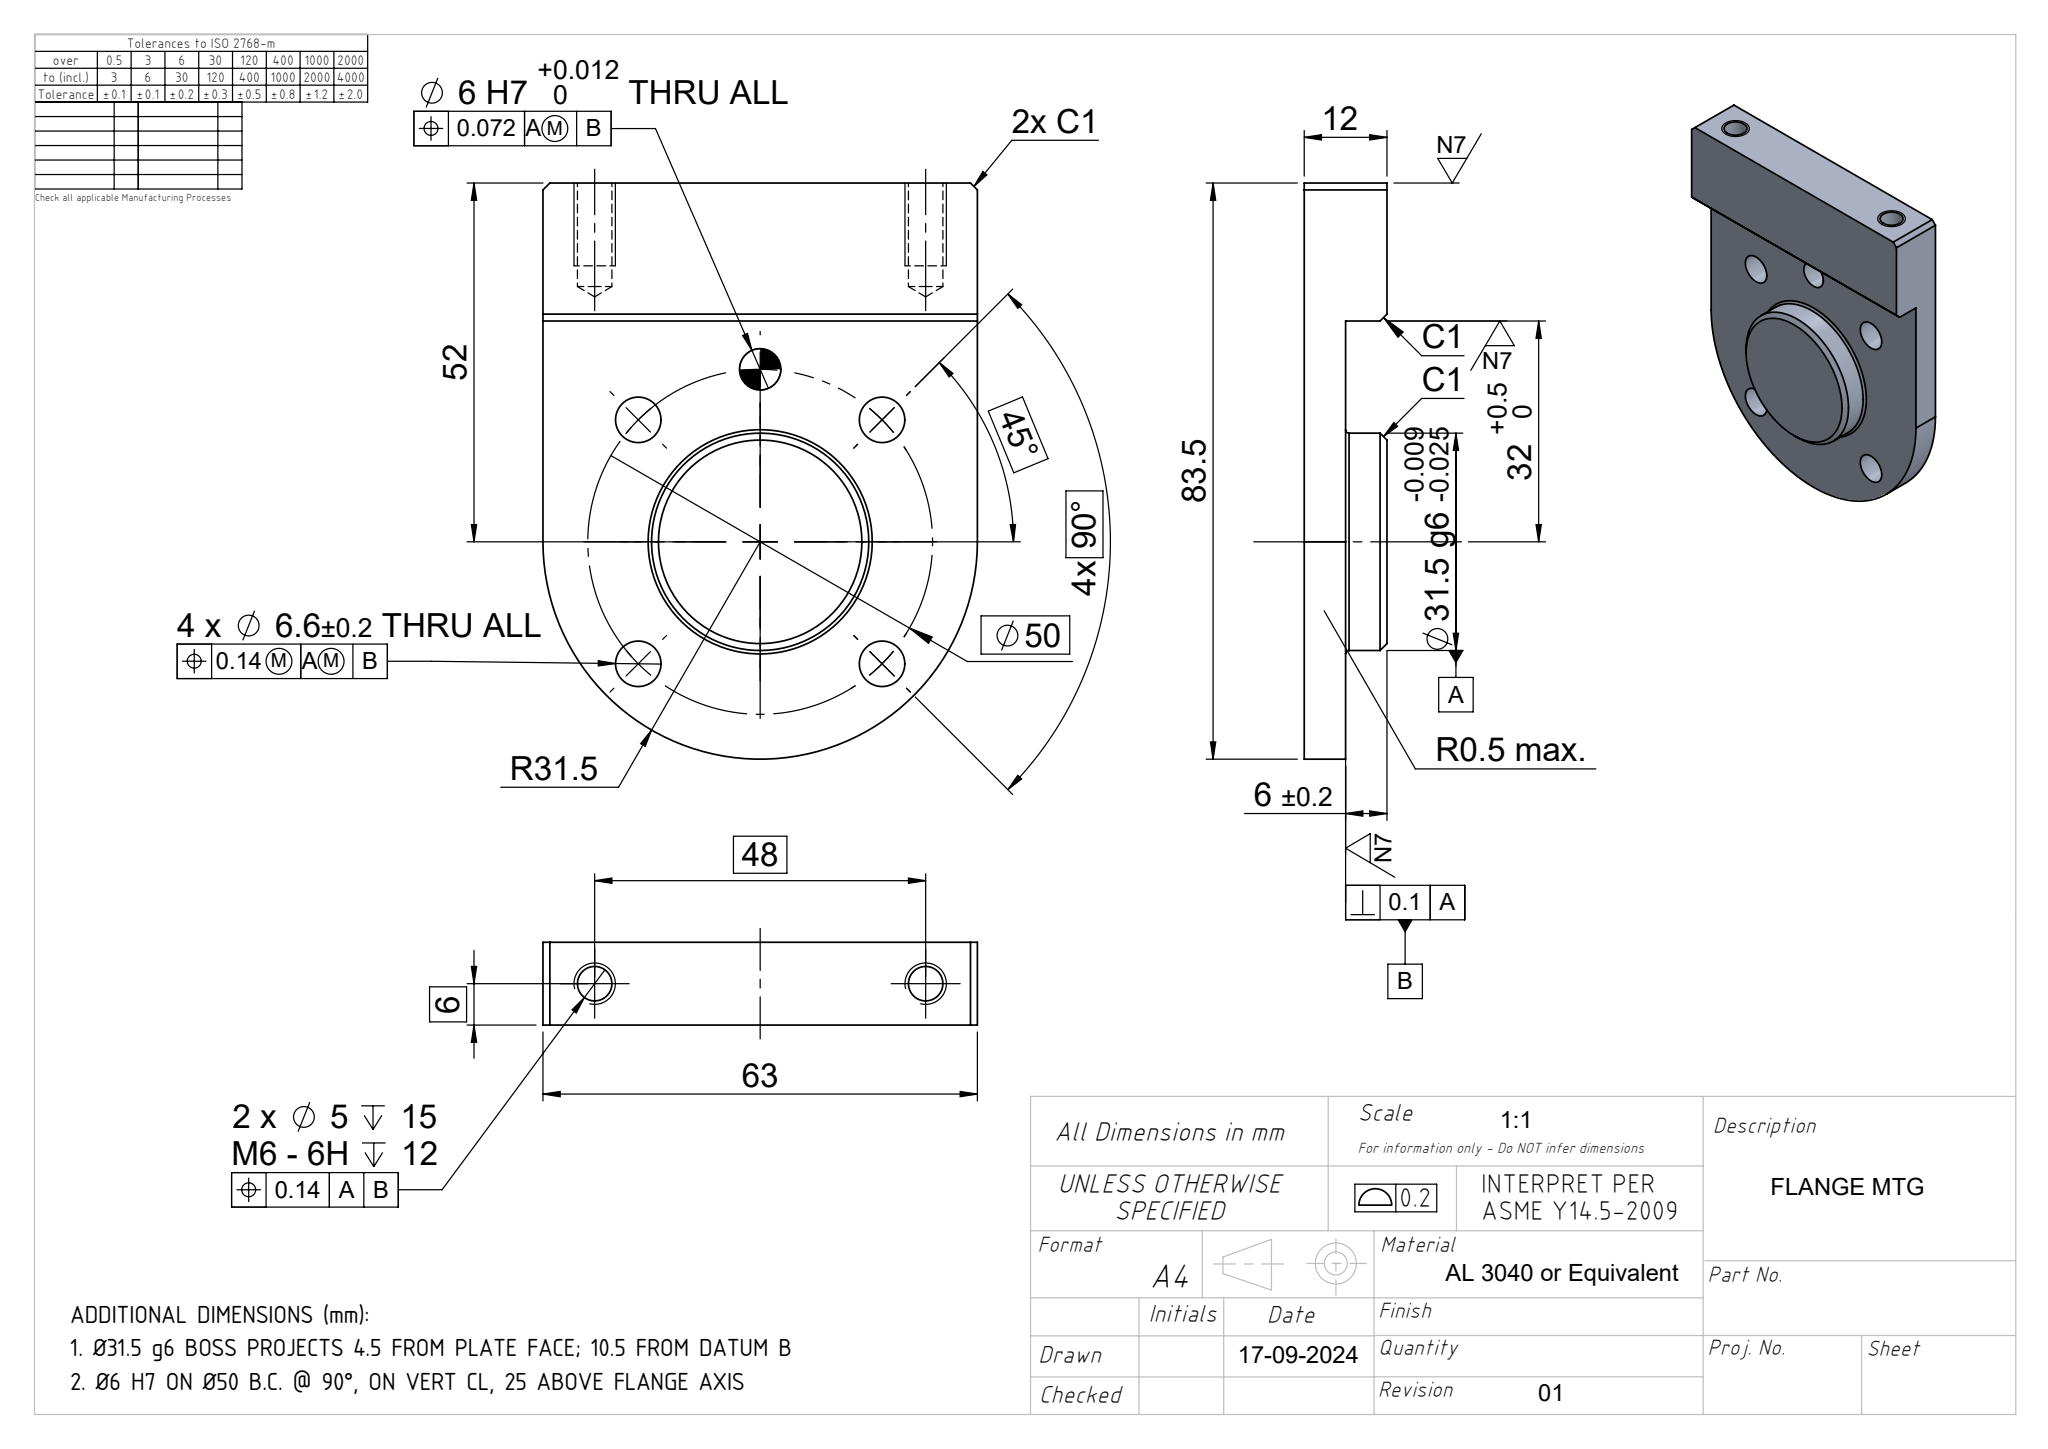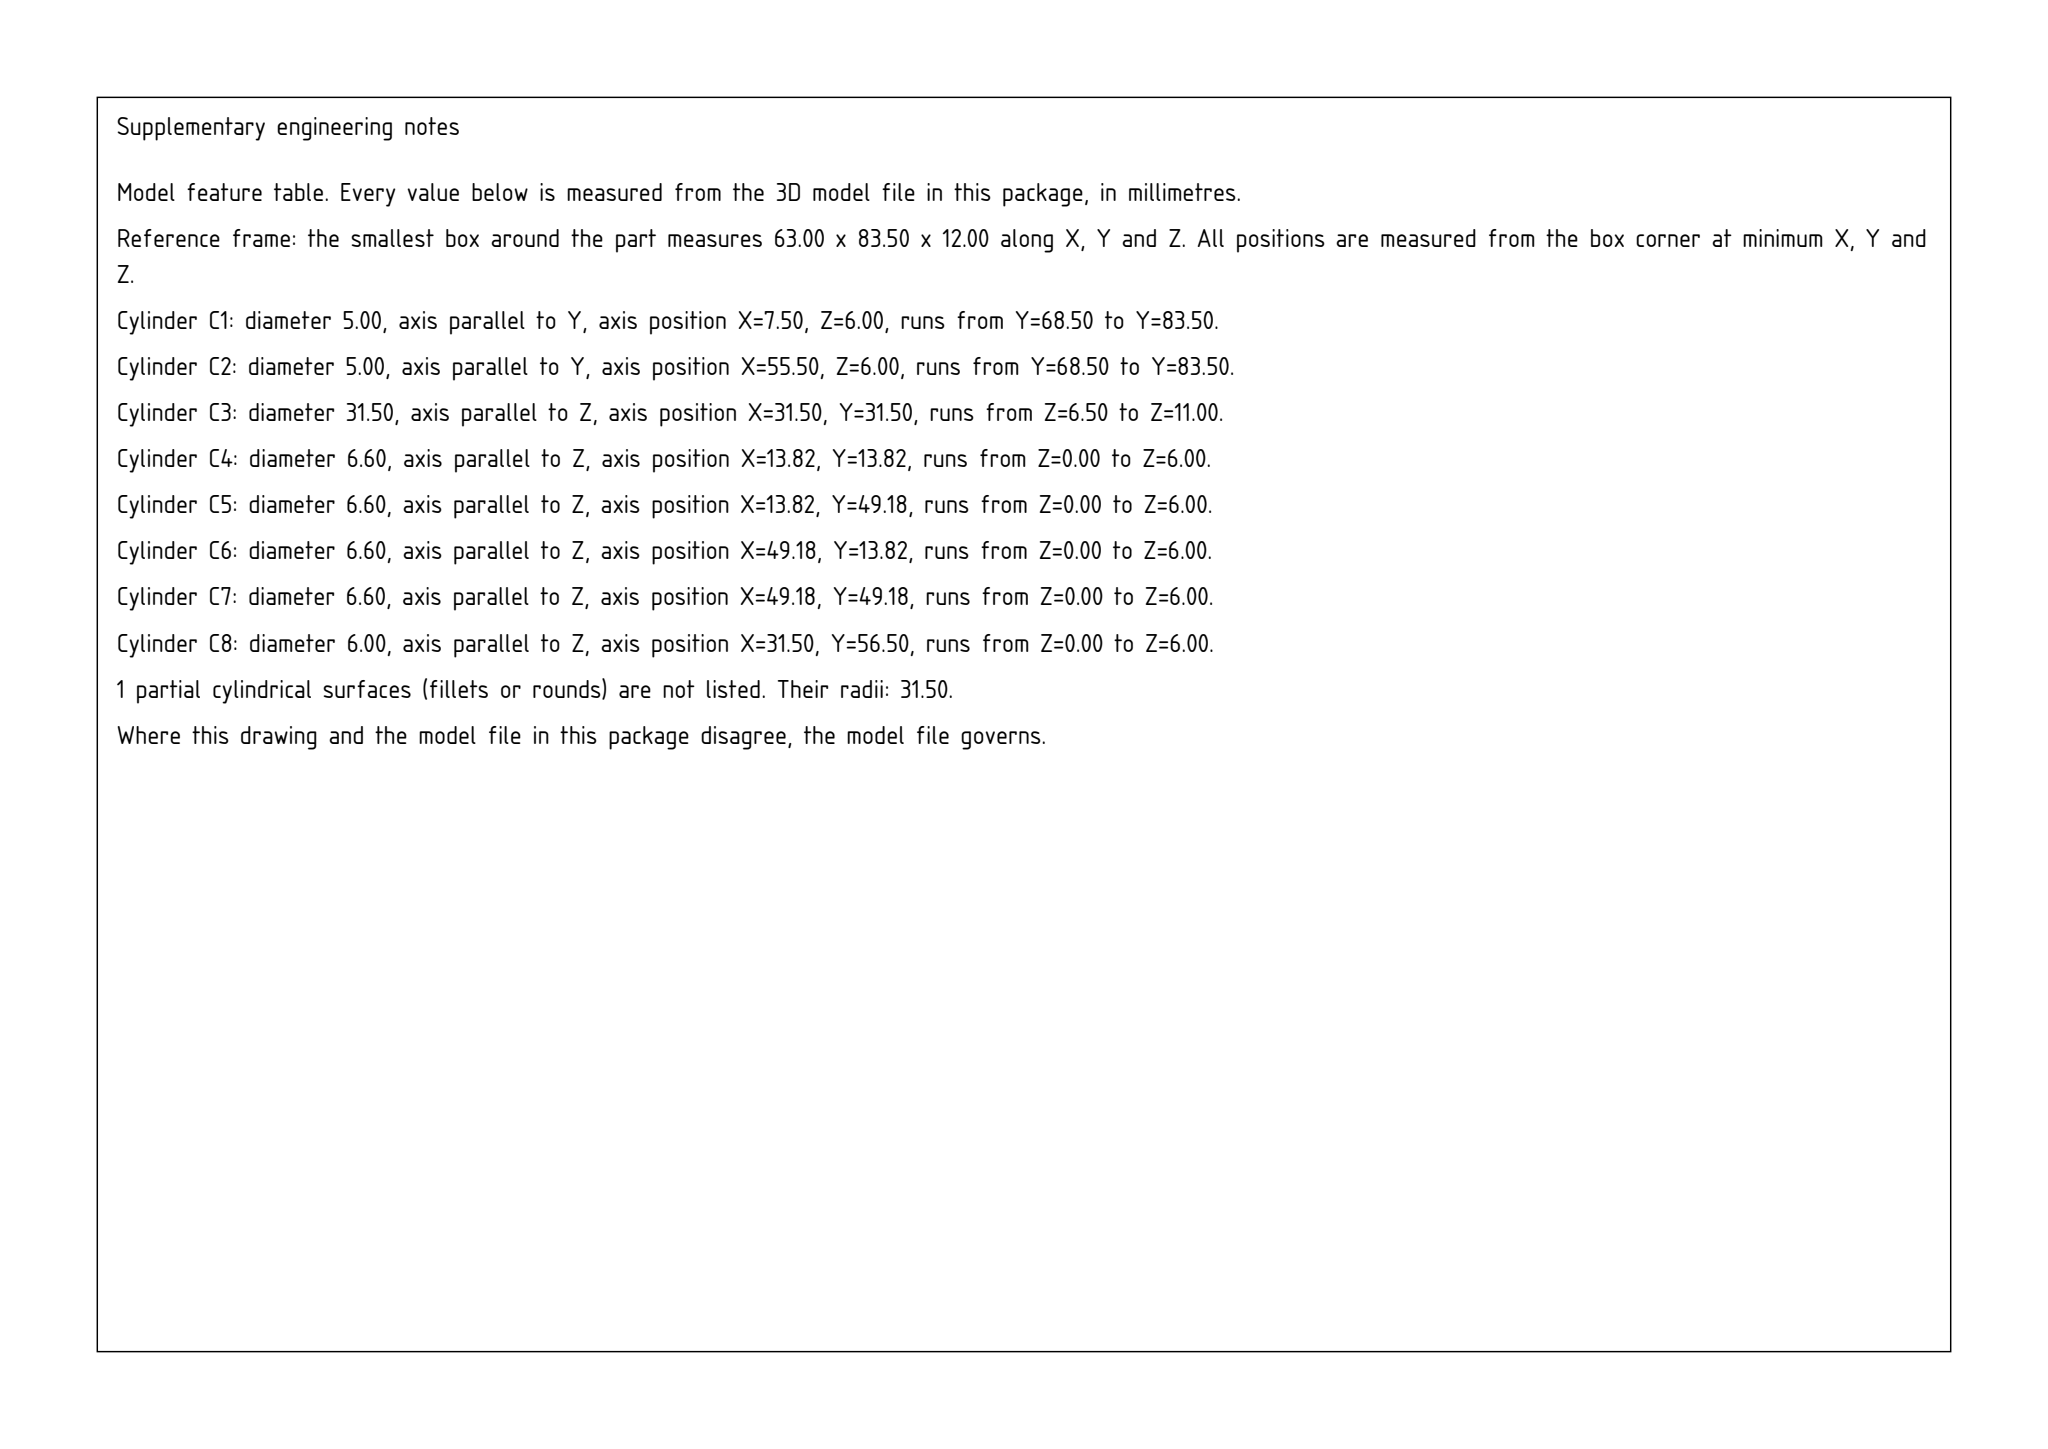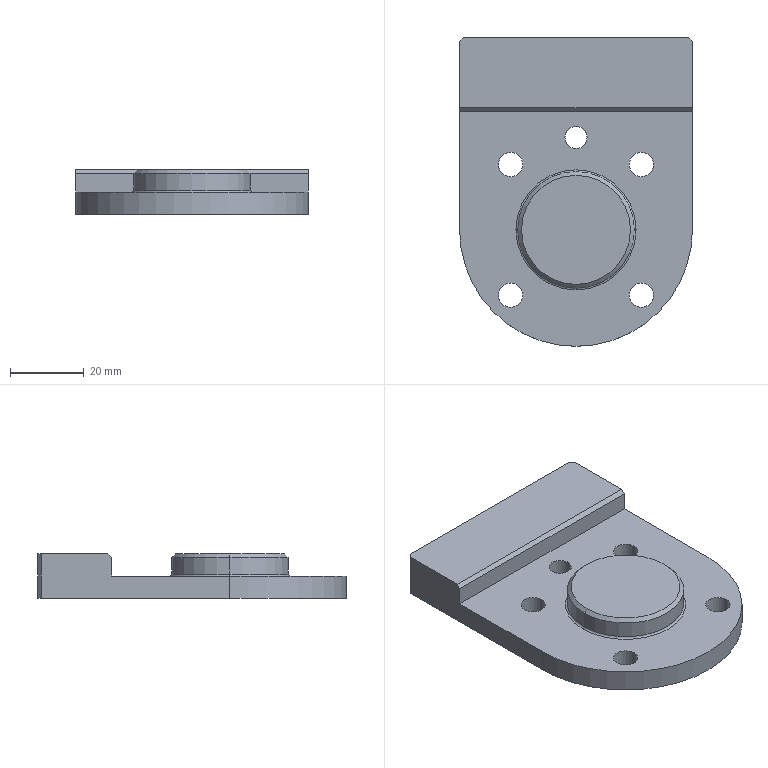Part | SolidWorks | mm | 1 solid | 36 faces | box 63 x 83.5 x 12 mm | volume 39558 mm3 | cylinder 17 | plane 11 | cone 6 | torus 2 | commonest cylinder face diameters 6.6 x8 5 x4 6 x2 31.5 x2 63 x1
build123d program:
from build123d import *

# Parameters (mm, degrees)
BOSS_EXTRUDE1_DEPTH   = 6
SKETCH2_R             = 15.75
BOSS_EXTRUDE2_DEPTH   = 6
CHAMFER1_SIZE         = 1
FILLET1_R             = 0.5
SKETCH12_W            = 63
SKETCH12_H            = 20
BOSS_EXTRUDE3_DEPTH   = 6
CHAMFER2_SIZE         = 1
M6_CLEARANCE_HOLE1_D  = 6.6
M6_TAPPED_HOLE1_D     = 5
M6_TAPPED_HOLE1_DEPTH = 15
M6_TAPPED_HOLE1_TIP   = 1.502
F_6_0MM_DOWEL_HOLE1_D = 6


with BuildPart() as part:
    # Sketch1 → Boss-Extrude1 (new body)
    with BuildSketch(Plane.XY):
        with BuildLine():
            Line((-31.5, 52), (31.5, 52))
            Line((31.5, 52), (31.5, 0))
            ThreePointArc((31.5, 0), (0, -31.5), (-31.5, 0))
            Line((-31.5, 0), (-31.5, 52))
        make_face()
    extrude(amount=BOSS_EXTRUDE1_DEPTH)

    # Sketch2 → Boss-Extrude2 (add)
    with BuildSketch(Plane.XY.offset(6)):
        Circle(SKETCH2_R)
    extrude(amount=BOSS_EXTRUDE2_DEPTH)

    # Chamfer1
    chamfer1_edges = [part.edges().sort_by_distance(p)[0] for p in [
        (-15.75, 0, 12),
    ]]
    chamfer(chamfer1_edges, length=CHAMFER1_SIZE)

    # Fillet1
    fillet1_edges = [part.edges().sort_by_distance(p)[0] for p in [
        (-15.75, 0, 6),
    ]]
    fillet(fillet1_edges, radius=FILLET1_R)

    # Sketch12 → Boss-Extrude3 (add)
    with BuildSketch(Plane.XY.offset(6)):
        with Locations((0, 42)):
            Rectangle(SKETCH12_W, SKETCH12_H)
    extrude(amount=BOSS_EXTRUDE3_DEPTH)

    # Chamfer2
    chamfer2_edges = [part.edges().sort_by_distance(p)[0] for p in [
        (0, 32, 12),
        (-31.5, 52, 6),
        (31.5, 52, 6),
    ]]
    chamfer(chamfer2_edges, length=CHAMFER2_SIZE)

    # M6 Clearance Hole1 (through all)
    with Locations(Plane(origin=(0, 0, 0), x_dir=(-1, 0, 0), z_dir=(0, 0, -1))):
        with Locations((17.678, 17.678), (-17.678, 17.678), (-17.678, -17.678), (17.678, -17.678)):
            Hole(M6_CLEARANCE_HOLE1_D / 2)

    # M6 Tapped Hole1
    with Locations(Plane(origin=(14.487, 52, 44.809), x_dir=(1, 0, 0), z_dir=(0, 1, 0))):
        with Locations((-38.487, 38.809), (9.513, 38.809)):
            Hole(M6_TAPPED_HOLE1_D / 2, depth=M6_TAPPED_HOLE1_DEPTH)
            with Locations((0, 0, -(M6_TAPPED_HOLE1_DEPTH + M6_TAPPED_HOLE1_TIP / 2))):  # 118° drill point
                Cone(0, M6_TAPPED_HOLE1_D / 2, M6_TAPPED_HOLE1_TIP, mode=Mode.SUBTRACT)

    # 6.0mm Dowel Hole1 (through all)
    with Locations(Plane(origin=(0, 0, 0), x_dir=(-1, 0, 0), z_dir=(0, 0, -1))):
        with Locations((0, 25)):
            Hole(F_6_0MM_DOWEL_HOLE1_D / 2)


solid = part.part